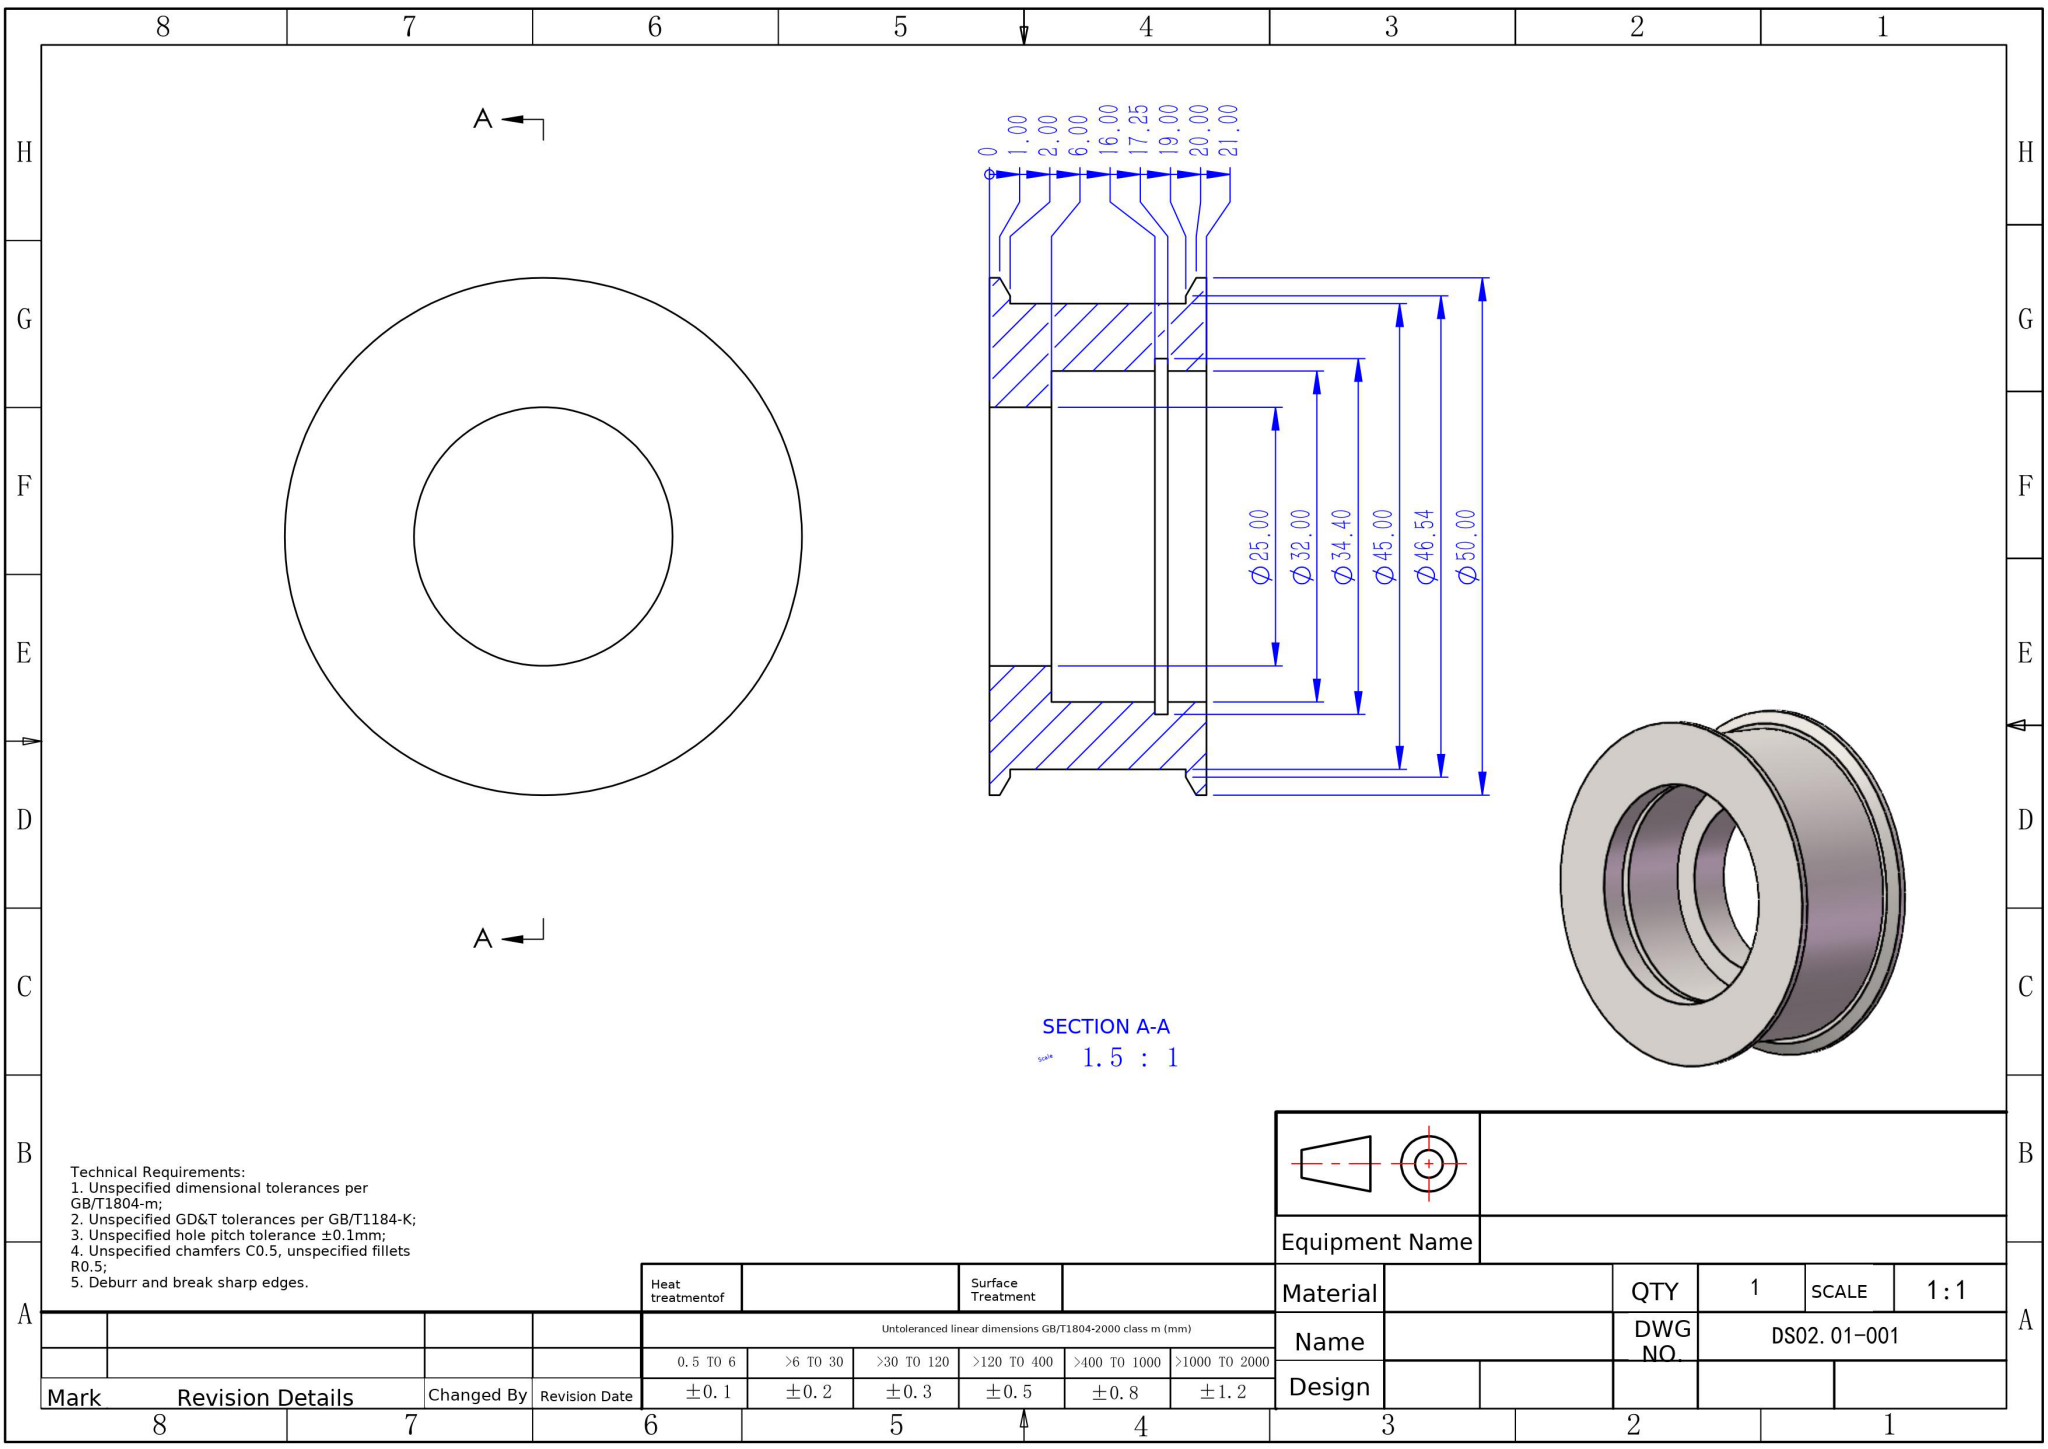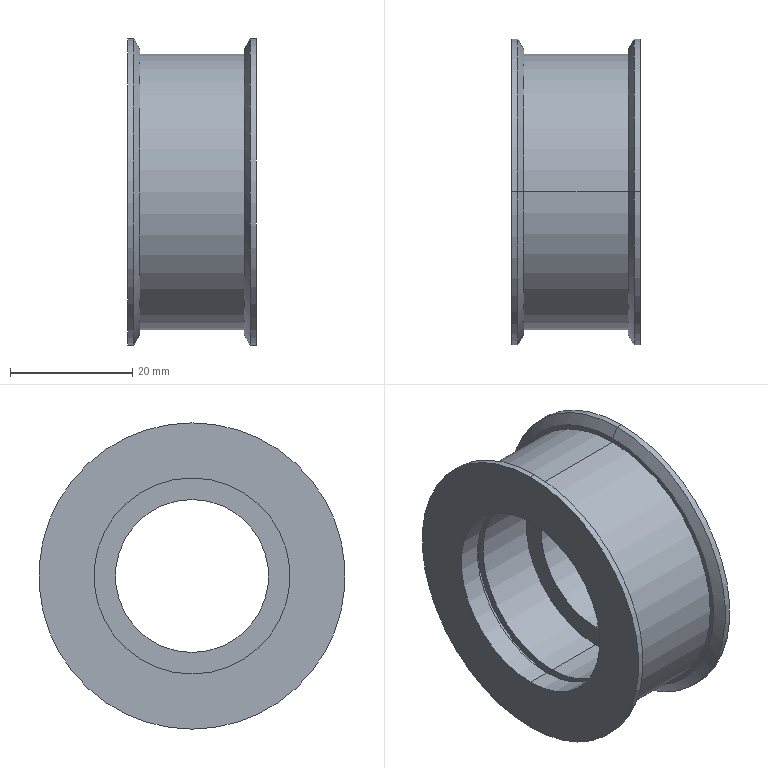Part | NX | mm | 1 solid | 25 faces | box 21 x 50 x 50 mm | volume 19460 mm3 | cylinder 14 | plane 7 | cone 4 | commonest cylinder face diameters 32 x4 50 x4 34.4 x2 45 x2 25 x2
STEP:
#1=CARTESIAN_POINT('',(-17.25,0.,17.2));
#2=VERTEX_POINT('',#1);
#3=CARTESIAN_POINT('',(-17.25,0.,-17.2));
#4=VERTEX_POINT('',#3);
#5=CARTESIAN_POINT('',(-17.25,0.,0.));
#6=DIRECTION('',(1.,0.,0.));
#7=DIRECTION('',(0.,0.,-1.));
#8=AXIS2_PLACEMENT_3D('',#5,#6,#7);
#9=CIRCLE('',#8,17.2);
#10=EDGE_CURVE('',#2,#4,#9,.T.);
#11=ORIENTED_EDGE('',*,*,#10,.F.);
#12=CARTESIAN_POINT('',(-16.,0.,17.2));
#13=VERTEX_POINT('',#12);
#14=CARTESIAN_POINT('',(0.,0.,17.2));
#15=DIRECTION('',(1.,0.,0.));
#16=VECTOR('',#15,1000.);
#17=LINE('',#14,#16);
#18=EDGE_CURVE('',#2,#13,#17,.T.);
#19=ORIENTED_EDGE('',*,*,#18,.T.);
#20=CARTESIAN_POINT('',(-16.,0.,-17.2));
#21=VERTEX_POINT('',#20);
#22=CARTESIAN_POINT('',(-16.,0.,0.));
#23=DIRECTION('',(1.,0.,0.));
#24=DIRECTION('',(0.,0.,-1.));
#25=AXIS2_PLACEMENT_3D('',#22,#23,#24);
#26=CIRCLE('',#25,17.2);
#27=EDGE_CURVE('',#13,#21,#26,.T.);
#28=ORIENTED_EDGE('',*,*,#27,.T.);
#29=CARTESIAN_POINT('',(0.,0.,-17.2));
#30=DIRECTION('',(1.,0.,0.));
#31=VECTOR('',#30,1000.);
#32=LINE('',#29,#31);
#33=EDGE_CURVE('',#4,#21,#32,.T.);
#34=ORIENTED_EDGE('',*,*,#33,.F.);
#35=EDGE_LOOP('',(#11,#19,#28,#34));
#36=FACE_OUTER_BOUND('',#35,.T.);
#37=CARTESIAN_POINT('',(0.,0.,0.));
#38=DIRECTION('',(1.,0.,0.));
#39=DIRECTION('',(0.,0.,-1.));
#40=AXIS2_PLACEMENT_3D('',#37,#38,#39);
#41=CYLINDRICAL_SURFACE('',#40,17.2);
#42=ADVANCED_FACE('',(#36),#41,.F.);
#43=CARTESIAN_POINT('',(-6.,0.,-16.));
#44=VERTEX_POINT('',#43);
#45=CARTESIAN_POINT('',(-6.,0.,16.));
#46=VERTEX_POINT('',#45);
#47=CARTESIAN_POINT('',(-6.,0.,0.));
#48=DIRECTION('',(-1.,0.,0.));
#49=DIRECTION('',(0.,0.,1.));
#50=AXIS2_PLACEMENT_3D('',#47,#48,#49);
#51=CIRCLE('',#50,16.);
#52=EDGE_CURVE('',#44,#46,#51,.T.);
#53=ORIENTED_EDGE('',*,*,#52,.F.);
#54=CARTESIAN_POINT('',(-16.,0.,-16.));
#55=VERTEX_POINT('',#54);
#56=CARTESIAN_POINT('',(-6.,0.,-16.));
#57=DIRECTION('',(-1.,0.,0.));
#58=VECTOR('',#57,1000.);
#59=LINE('',#56,#58);
#60=EDGE_CURVE('',#44,#55,#59,.T.);
#61=ORIENTED_EDGE('',*,*,#60,.T.);
#62=CARTESIAN_POINT('',(-16.,0.,16.));
#63=VERTEX_POINT('',#62);
#64=CARTESIAN_POINT('',(-16.,0.,0.));
#65=DIRECTION('',(1.,0.,0.));
#66=DIRECTION('',(0.,0.,-1.));
#67=AXIS2_PLACEMENT_3D('',#64,#65,#66);
#68=CIRCLE('',#67,16.);
#69=EDGE_CURVE('',#63,#55,#68,.T.);
#70=ORIENTED_EDGE('',*,*,#69,.F.);
#71=CARTESIAN_POINT('',(-6.,0.,16.));
#72=DIRECTION('',(-1.,0.,0.));
#73=VECTOR('',#72,1000.);
#74=LINE('',#71,#73);
#75=EDGE_CURVE('',#46,#63,#74,.T.);
#76=ORIENTED_EDGE('',*,*,#75,.F.);
#77=EDGE_LOOP('',(#53,#61,#70,#76));
#78=FACE_OUTER_BOUND('',#77,.T.);
#79=CARTESIAN_POINT('',(-6.,0.,0.));
#80=DIRECTION('',(-1.,0.,0.));
#81=DIRECTION('',(0.,0.,1.));
#82=AXIS2_PLACEMENT_3D('',#79,#80,#81);
#83=CYLINDRICAL_SURFACE('',#82,16.);
#84=ADVANCED_FACE('',(#78),#83,.F.);
#85=CARTESIAN_POINT('',(-21.,0.,-25.));
#86=VERTEX_POINT('',#85);
#87=CARTESIAN_POINT('',(-21.,0.,25.));
#88=VERTEX_POINT('',#87);
#89=CARTESIAN_POINT('',(-21.,0.,0.));
#90=DIRECTION('',(1.,0.,0.));
#91=DIRECTION('',(0.,0.,-1.));
#92=AXIS2_PLACEMENT_3D('',#89,#90,#91);
#93=CIRCLE('',#92,25.);
#94=EDGE_CURVE('',#86,#88,#93,.T.);
#95=ORIENTED_EDGE('',*,*,#94,.T.);
#96=CARTESIAN_POINT('',(-20.,0.,25.));
#97=VERTEX_POINT('',#96);
#98=CARTESIAN_POINT('',(0.,0.,25.));
#99=DIRECTION('',(1.,0.,0.));
#100=VECTOR('',#99,1000.);
#101=LINE('',#98,#100);
#102=EDGE_CURVE('',#88,#97,#101,.T.);
#103=ORIENTED_EDGE('',*,*,#102,.T.);
#104=CARTESIAN_POINT('',(-20.,0.,-25.));
#105=VERTEX_POINT('',#104);
#106=CARTESIAN_POINT('',(-20.,0.,0.));
#107=DIRECTION('',(1.,0.,0.));
#108=DIRECTION('',(0.,0.,-1.));
#109=AXIS2_PLACEMENT_3D('',#106,#107,#108);
#110=CIRCLE('',#109,25.);
#111=EDGE_CURVE('',#105,#97,#110,.T.);
#112=ORIENTED_EDGE('',*,*,#111,.F.);
#113=CARTESIAN_POINT('',(0.,0.,-25.));
#114=DIRECTION('',(1.,0.,0.));
#115=VECTOR('',#114,1000.);
#116=LINE('',#113,#115);
#117=EDGE_CURVE('',#86,#105,#116,.T.);
#118=ORIENTED_EDGE('',*,*,#117,.F.);
#119=EDGE_LOOP('',(#95,#103,#112,#118));
#120=FACE_OUTER_BOUND('',#119,.T.);
#121=CARTESIAN_POINT('',(0.,0.,0.));
#122=DIRECTION('',(1.,0.,0.));
#123=DIRECTION('',(0.,0.,-1.));
#124=AXIS2_PLACEMENT_3D('',#121,#122,#123);
#125=CYLINDRICAL_SURFACE('',#124,25.);
#126=ADVANCED_FACE('',(#120),#125,.T.);
#127=CARTESIAN_POINT('',(-19.,0.,-23.268));
#128=VERTEX_POINT('',#127);
#129=CARTESIAN_POINT('',(-19.,0.,23.268));
#130=VERTEX_POINT('',#129);
#131=CARTESIAN_POINT('',(-19.,0.,0.));
#132=DIRECTION('',(1.,0.,0.));
#133=DIRECTION('',(0.,0.,-1.));
#134=AXIS2_PLACEMENT_3D('',#131,#132,#133);
#135=CIRCLE('',#134,23.268);
#136=EDGE_CURVE('',#128,#130,#135,.T.);
#137=ORIENTED_EDGE('',*,*,#136,.F.);
#138=CARTESIAN_POINT('',(-19.,0.,-23.268));
#139=DIRECTION('',(-0.5,0.,-0.866));
#140=VECTOR('',#139,1000.);
#141=LINE('',#138,#140);
#142=EDGE_CURVE('',#128,#105,#141,.T.);
#143=ORIENTED_EDGE('',*,*,#142,.T.);
#144=ORIENTED_EDGE('',*,*,#111,.T.);
#145=CARTESIAN_POINT('',(-19.,0.,23.268));
#146=DIRECTION('',(-0.5,0.,0.866));
#147=VECTOR('',#146,1000.);
#148=LINE('',#145,#147);
#149=EDGE_CURVE('',#130,#97,#148,.T.);
#150=ORIENTED_EDGE('',*,*,#149,.F.);
#151=EDGE_LOOP('',(#137,#143,#144,#150));
#152=FACE_OUTER_BOUND('',#151,.T.);
#153=CARTESIAN_POINT('',(-19.,0.,0.));
#154=DIRECTION('',(-1.,0.,0.));
#155=DIRECTION('',(0.,0.,1.));
#156=AXIS2_PLACEMENT_3D('',#153,#154,#155);
#157=CONICAL_SURFACE('',#156,23.268,1.047);
#158=ADVANCED_FACE('',(#152),#157,.T.);
#159=CARTESIAN_POINT('',(-19.,0.,-22.5));
#160=VERTEX_POINT('',#159);
#161=CARTESIAN_POINT('',(-19.,0.,22.5));
#162=VERTEX_POINT('',#161);
#163=CARTESIAN_POINT('',(-19.,0.,0.));
#164=DIRECTION('',(1.,0.,0.));
#165=DIRECTION('',(0.,0.,-1.));
#166=AXIS2_PLACEMENT_3D('',#163,#164,#165);
#167=CIRCLE('',#166,22.5);
#168=EDGE_CURVE('',#160,#162,#167,.T.);
#169=ORIENTED_EDGE('',*,*,#168,.T.);
#170=CARTESIAN_POINT('',(-2.,0.,22.5));
#171=VERTEX_POINT('',#170);
#172=CARTESIAN_POINT('',(0.,0.,22.5));
#173=DIRECTION('',(1.,0.,0.));
#174=VECTOR('',#173,1000.);
#175=LINE('',#172,#174);
#176=EDGE_CURVE('',#162,#171,#175,.T.);
#177=ORIENTED_EDGE('',*,*,#176,.T.);
#178=CARTESIAN_POINT('',(-2.,0.,-22.5));
#179=VERTEX_POINT('',#178);
#180=CARTESIAN_POINT('',(-2.,0.,0.));
#181=DIRECTION('',(1.,0.,0.));
#182=DIRECTION('',(0.,0.,-1.));
#183=AXIS2_PLACEMENT_3D('',#180,#181,#182);
#184=CIRCLE('',#183,22.5);
#185=EDGE_CURVE('',#179,#171,#184,.T.);
#186=ORIENTED_EDGE('',*,*,#185,.F.);
#187=CARTESIAN_POINT('',(0.,0.,-22.5));
#188=DIRECTION('',(1.,0.,0.));
#189=VECTOR('',#188,1000.);
#190=LINE('',#187,#189);
#191=EDGE_CURVE('',#160,#179,#190,.T.);
#192=ORIENTED_EDGE('',*,*,#191,.F.);
#193=EDGE_LOOP('',(#169,#177,#186,#192));
#194=FACE_OUTER_BOUND('',#193,.T.);
#195=CARTESIAN_POINT('',(0.,0.,0.));
#196=DIRECTION('',(1.,0.,0.));
#197=DIRECTION('',(0.,0.,-1.));
#198=AXIS2_PLACEMENT_3D('',#195,#196,#197);
#199=CYLINDRICAL_SURFACE('',#198,22.5);
#200=ADVANCED_FACE('',(#194),#199,.T.);
#201=CARTESIAN_POINT('',(-2.,0.,-23.268));
#202=VERTEX_POINT('',#201);
#203=CARTESIAN_POINT('',(-2.,0.,23.268));
#204=VERTEX_POINT('',#203);
#205=CARTESIAN_POINT('',(-2.,0.,0.));
#206=DIRECTION('',(1.,0.,0.));
#207=DIRECTION('',(0.,0.,-1.));
#208=AXIS2_PLACEMENT_3D('',#205,#206,#207);
#209=CIRCLE('',#208,23.268);
#210=EDGE_CURVE('',#202,#204,#209,.T.);
#211=ORIENTED_EDGE('',*,*,#210,.T.);
#212=CARTESIAN_POINT('',(-1.,0.,25.));
#213=VERTEX_POINT('',#212);
#214=CARTESIAN_POINT('',(-1.,0.,25.));
#215=DIRECTION('',(0.5,0.,0.866));
#216=VECTOR('',#215,1000.);
#217=LINE('',#214,#216);
#218=EDGE_CURVE('',#204,#213,#217,.T.);
#219=ORIENTED_EDGE('',*,*,#218,.T.);
#220=CARTESIAN_POINT('',(-1.,0.,-25.));
#221=VERTEX_POINT('',#220);
#222=CARTESIAN_POINT('',(-1.,0.,0.));
#223=DIRECTION('',(1.,0.,0.));
#224=DIRECTION('',(0.,0.,-1.));
#225=AXIS2_PLACEMENT_3D('',#222,#223,#224);
#226=CIRCLE('',#225,25.);
#227=EDGE_CURVE('',#221,#213,#226,.T.);
#228=ORIENTED_EDGE('',*,*,#227,.F.);
#229=CARTESIAN_POINT('',(-1.,0.,-25.));
#230=DIRECTION('',(0.5,0.,-0.866));
#231=VECTOR('',#230,1000.);
#232=LINE('',#229,#231);
#233=EDGE_CURVE('',#202,#221,#232,.T.);
#234=ORIENTED_EDGE('',*,*,#233,.F.);
#235=EDGE_LOOP('',(#211,#219,#228,#234));
#236=FACE_OUTER_BOUND('',#235,.T.);
#237=CARTESIAN_POINT('',(-1.,0.,0.));
#238=DIRECTION('',(1.,0.,0.));
#239=DIRECTION('',(0.,0.,-1.));
#240=AXIS2_PLACEMENT_3D('',#237,#238,#239);
#241=CONICAL_SURFACE('',#240,25.,1.047);
#242=ADVANCED_FACE('',(#236),#241,.T.);
#243=ORIENTED_EDGE('',*,*,#227,.T.);
#244=CARTESIAN_POINT('',(-0.,0.,25.));
#245=VERTEX_POINT('',#244);
#246=CARTESIAN_POINT('',(0.,0.,25.));
#247=DIRECTION('',(1.,0.,0.));
#248=VECTOR('',#247,1000.);
#249=LINE('',#246,#248);
#250=EDGE_CURVE('',#213,#245,#249,.T.);
#251=ORIENTED_EDGE('',*,*,#250,.T.);
#252=CARTESIAN_POINT('',(-0.,0.,-25.));
#253=VERTEX_POINT('',#252);
#254=CARTESIAN_POINT('',(-0.,0.,0.));
#255=DIRECTION('',(1.,0.,0.));
#256=DIRECTION('',(0.,0.,-1.));
#257=AXIS2_PLACEMENT_3D('',#254,#255,#256);
#258=CIRCLE('',#257,25.);
#259=EDGE_CURVE('',#253,#245,#258,.T.);
#260=ORIENTED_EDGE('',*,*,#259,.F.);
#261=CARTESIAN_POINT('',(0.,0.,-25.));
#262=DIRECTION('',(1.,0.,0.));
#263=VECTOR('',#262,1000.);
#264=LINE('',#261,#263);
#265=EDGE_CURVE('',#221,#253,#264,.T.);
#266=ORIENTED_EDGE('',*,*,#265,.F.);
#267=EDGE_LOOP('',(#243,#251,#260,#266));
#268=FACE_OUTER_BOUND('',#267,.T.);
#269=CARTESIAN_POINT('',(0.,0.,0.));
#270=DIRECTION('',(1.,0.,0.));
#271=DIRECTION('',(0.,0.,-1.));
#272=AXIS2_PLACEMENT_3D('',#269,#270,#271);
#273=CYLINDRICAL_SURFACE('',#272,25.);
#274=ADVANCED_FACE('',(#268),#273,.T.);
#275=CARTESIAN_POINT('',(-6.,0.,-12.5));
#276=VERTEX_POINT('',#275);
#277=CARTESIAN_POINT('',(-6.,0.,12.5));
#278=VERTEX_POINT('',#277);
#279=CARTESIAN_POINT('',(-6.,0.,0.));
#280=DIRECTION('',(-1.,0.,0.));
#281=DIRECTION('',(0.,0.,1.));
#282=AXIS2_PLACEMENT_3D('',#279,#280,#281);
#283=CIRCLE('',#282,12.5);
#284=EDGE_CURVE('',#276,#278,#283,.T.);
#285=ORIENTED_EDGE('',*,*,#284,.T.);
#286=CARTESIAN_POINT('',(0.,0.,12.5));
#287=VERTEX_POINT('',#286);
#288=CARTESIAN_POINT('',(0.,0.,12.5));
#289=DIRECTION('',(1.,0.,0.));
#290=VECTOR('',#289,1000.);
#291=LINE('',#288,#290);
#292=EDGE_CURVE('',#278,#287,#291,.T.);
#293=ORIENTED_EDGE('',*,*,#292,.T.);
#294=CARTESIAN_POINT('',(0.,0.,-12.5));
#295=VERTEX_POINT('',#294);
#296=CARTESIAN_POINT('',(0.,0.,0.));
#297=DIRECTION('',(1.,0.,0.));
#298=DIRECTION('',(0.,0.,-1.));
#299=AXIS2_PLACEMENT_3D('',#296,#297,#298);
#300=CIRCLE('',#299,12.5);
#301=EDGE_CURVE('',#287,#295,#300,.T.);
#302=ORIENTED_EDGE('',*,*,#301,.T.);
#303=CARTESIAN_POINT('',(0.,0.,-12.5));
#304=DIRECTION('',(1.,0.,0.));
#305=VECTOR('',#304,1000.);
#306=LINE('',#303,#305);
#307=EDGE_CURVE('',#276,#295,#306,.T.);
#308=ORIENTED_EDGE('',*,*,#307,.F.);
#309=EDGE_LOOP('',(#285,#293,#302,#308));
#310=FACE_OUTER_BOUND('',#309,.T.);
#311=CARTESIAN_POINT('',(0.,0.,0.));
#312=DIRECTION('',(1.,0.,0.));
#313=DIRECTION('',(0.,0.,-1.));
#314=AXIS2_PLACEMENT_3D('',#311,#312,#313);
#315=CYLINDRICAL_SURFACE('',#314,12.5);
#316=ADVANCED_FACE('',(#310),#315,.F.);
#317=CARTESIAN_POINT('',(-17.25,0.,16.));
#318=VERTEX_POINT('',#317);
#319=CARTESIAN_POINT('',(-17.25,0.,-16.));
#320=VERTEX_POINT('',#319);
#321=CARTESIAN_POINT('',(-17.25,0.,0.));
#322=DIRECTION('',(1.,0.,0.));
#323=DIRECTION('',(0.,0.,-1.));
#324=AXIS2_PLACEMENT_3D('',#321,#322,#323);
#325=CIRCLE('',#324,16.);
#326=EDGE_CURVE('',#318,#320,#325,.T.);
#327=ORIENTED_EDGE('',*,*,#326,.T.);
#328=CARTESIAN_POINT('',(-21.,0.,-16.));
#329=VERTEX_POINT('',#328);
#330=CARTESIAN_POINT('',(-6.,0.,-16.));
#331=DIRECTION('',(-1.,0.,0.));
#332=VECTOR('',#331,1000.);
#333=LINE('',#330,#332);
#334=EDGE_CURVE('',#320,#329,#333,.T.);
#335=ORIENTED_EDGE('',*,*,#334,.T.);
#336=CARTESIAN_POINT('',(-21.,0.,16.));
#337=VERTEX_POINT('',#336);
#338=CARTESIAN_POINT('',(-21.,0.,0.));
#339=DIRECTION('',(-1.,0.,0.));
#340=DIRECTION('',(0.,0.,1.));
#341=AXIS2_PLACEMENT_3D('',#338,#339,#340);
#342=CIRCLE('',#341,16.);
#343=EDGE_CURVE('',#329,#337,#342,.T.);
#344=ORIENTED_EDGE('',*,*,#343,.T.);
#345=CARTESIAN_POINT('',(-6.,0.,16.));
#346=DIRECTION('',(-1.,0.,0.));
#347=VECTOR('',#346,1000.);
#348=LINE('',#345,#347);
#349=EDGE_CURVE('',#318,#337,#348,.T.);
#350=ORIENTED_EDGE('',*,*,#349,.F.);
#351=EDGE_LOOP('',(#327,#335,#344,#350));
#352=FACE_OUTER_BOUND('',#351,.T.);
#353=CARTESIAN_POINT('',(-6.,0.,0.));
#354=DIRECTION('',(-1.,0.,0.));
#355=DIRECTION('',(0.,0.,1.));
#356=AXIS2_PLACEMENT_3D('',#353,#354,#355);
#357=CYLINDRICAL_SURFACE('',#356,16.);
#358=ADVANCED_FACE('',(#352),#357,.F.);
#359=ORIENTED_EDGE('',*,*,#334,.F.);
#360=CARTESIAN_POINT('',(-17.25,0.,0.));
#361=DIRECTION('',(1.,0.,0.));
#362=DIRECTION('',(0.,0.,-1.));
#363=AXIS2_PLACEMENT_3D('',#360,#361,#362);
#364=CIRCLE('',#363,16.);
#365=EDGE_CURVE('',#320,#318,#364,.T.);
#366=ORIENTED_EDGE('',*,*,#365,.T.);
#367=ORIENTED_EDGE('',*,*,#349,.T.);
#368=CARTESIAN_POINT('',(-21.,0.,0.));
#369=DIRECTION('',(-1.,0.,0.));
#370=DIRECTION('',(0.,0.,1.));
#371=AXIS2_PLACEMENT_3D('',#368,#369,#370);
#372=CIRCLE('',#371,16.);
#373=EDGE_CURVE('',#337,#329,#372,.T.);
#374=ORIENTED_EDGE('',*,*,#373,.T.);
#375=EDGE_LOOP('',(#359,#366,#367,#374));
#376=FACE_OUTER_BOUND('',#375,.T.);
#377=CARTESIAN_POINT('',(-6.,0.,0.));
#378=DIRECTION('',(-1.,0.,0.));
#379=DIRECTION('',(0.,0.,1.));
#380=AXIS2_PLACEMENT_3D('',#377,#378,#379);
#381=CYLINDRICAL_SURFACE('',#380,16.);
#382=ADVANCED_FACE('',(#376),#381,.F.);
#383=ORIENTED_EDGE('',*,*,#292,.F.);
#384=CARTESIAN_POINT('',(-6.,0.,0.));
#385=DIRECTION('',(-1.,0.,0.));
#386=DIRECTION('',(0.,0.,1.));
#387=AXIS2_PLACEMENT_3D('',#384,#385,#386);
#388=CIRCLE('',#387,12.5);
#389=EDGE_CURVE('',#278,#276,#388,.T.);
#390=ORIENTED_EDGE('',*,*,#389,.T.);
#391=ORIENTED_EDGE('',*,*,#307,.T.);
#392=CARTESIAN_POINT('',(0.,0.,0.));
#393=DIRECTION('',(1.,0.,0.));
#394=DIRECTION('',(0.,0.,-1.));
#395=AXIS2_PLACEMENT_3D('',#392,#393,#394);
#396=CIRCLE('',#395,12.5);
#397=EDGE_CURVE('',#295,#287,#396,.T.);
#398=ORIENTED_EDGE('',*,*,#397,.T.);
#399=EDGE_LOOP('',(#383,#390,#391,#398));
#400=FACE_OUTER_BOUND('',#399,.T.);
#401=CARTESIAN_POINT('',(0.,0.,0.));
#402=DIRECTION('',(1.,0.,0.));
#403=DIRECTION('',(0.,0.,-1.));
#404=AXIS2_PLACEMENT_3D('',#401,#402,#403);
#405=CYLINDRICAL_SURFACE('',#404,12.5);
#406=ADVANCED_FACE('',(#400),#405,.F.);
#407=ORIENTED_EDGE('',*,*,#259,.T.);
#408=CARTESIAN_POINT('',(-0.,0.,0.));
#409=DIRECTION('',(1.,0.,0.));
#410=DIRECTION('',(0.,0.,-1.));
#411=AXIS2_PLACEMENT_3D('',#408,#409,#410);
#412=CIRCLE('',#411,25.);
#413=EDGE_CURVE('',#245,#253,#412,.T.);
#414=ORIENTED_EDGE('',*,*,#413,.T.);
#415=EDGE_LOOP('',(#407,#414));
#416=FACE_OUTER_BOUND('',#415,.T.);
#417=ORIENTED_EDGE('',*,*,#397,.F.);
#418=ORIENTED_EDGE('',*,*,#301,.F.);
#419=EDGE_LOOP('',(#417,#418));
#420=FACE_BOUND('',#419,.T.);
#421=CARTESIAN_POINT('',(-0.,12.5,0.));
#422=DIRECTION('',(1.,0.,0.));
#423=DIRECTION('',(0.,0.,-1.));
#424=AXIS2_PLACEMENT_3D('',#421,#422,#423);
#425=PLANE('',#424);
#426=ADVANCED_FACE('',(#416,#420),#425,.T.);
#427=ORIENTED_EDGE('',*,*,#250,.F.);
#428=CARTESIAN_POINT('',(-1.,0.,0.));
#429=DIRECTION('',(1.,0.,0.));
#430=DIRECTION('',(0.,0.,-1.));
#431=AXIS2_PLACEMENT_3D('',#428,#429,#430);
#432=CIRCLE('',#431,25.);
#433=EDGE_CURVE('',#213,#221,#432,.T.);
#434=ORIENTED_EDGE('',*,*,#433,.T.);
#435=ORIENTED_EDGE('',*,*,#265,.T.);
#436=ORIENTED_EDGE('',*,*,#413,.F.);
#437=EDGE_LOOP('',(#427,#434,#435,#436));
#438=FACE_OUTER_BOUND('',#437,.T.);
#439=CARTESIAN_POINT('',(0.,0.,0.));
#440=DIRECTION('',(1.,0.,0.));
#441=DIRECTION('',(0.,0.,-1.));
#442=AXIS2_PLACEMENT_3D('',#439,#440,#441);
#443=CYLINDRICAL_SURFACE('',#442,25.);
#444=ADVANCED_FACE('',(#438),#443,.T.);
#445=ORIENTED_EDGE('',*,*,#218,.F.);
#446=CARTESIAN_POINT('',(-2.,0.,0.));
#447=DIRECTION('',(1.,0.,0.));
#448=DIRECTION('',(0.,0.,-1.));
#449=AXIS2_PLACEMENT_3D('',#446,#447,#448);
#450=CIRCLE('',#449,23.268);
#451=EDGE_CURVE('',#204,#202,#450,.T.);
#452=ORIENTED_EDGE('',*,*,#451,.T.);
#453=ORIENTED_EDGE('',*,*,#233,.T.);
#454=ORIENTED_EDGE('',*,*,#433,.F.);
#455=EDGE_LOOP('',(#445,#452,#453,#454));
#456=FACE_OUTER_BOUND('',#455,.T.);
#457=CARTESIAN_POINT('',(-1.,0.,0.));
#458=DIRECTION('',(1.,0.,0.));
#459=DIRECTION('',(0.,0.,-1.));
#460=AXIS2_PLACEMENT_3D('',#457,#458,#459);
#461=CONICAL_SURFACE('',#460,25.,1.047);
#462=ADVANCED_FACE('',(#456),#461,.T.);
#463=ORIENTED_EDGE('',*,*,#185,.T.);
#464=CARTESIAN_POINT('',(-2.,0.,0.));
#465=DIRECTION('',(1.,0.,0.));
#466=DIRECTION('',(0.,0.,-1.));
#467=AXIS2_PLACEMENT_3D('',#464,#465,#466);
#468=CIRCLE('',#467,22.5);
#469=EDGE_CURVE('',#171,#179,#468,.T.);
#470=ORIENTED_EDGE('',*,*,#469,.T.);
#471=EDGE_LOOP('',(#463,#470));
#472=FACE_BOUND('',#471,.T.);
#473=ORIENTED_EDGE('',*,*,#210,.F.);
#474=ORIENTED_EDGE('',*,*,#451,.F.);
#475=EDGE_LOOP('',(#473,#474));
#476=FACE_OUTER_BOUND('',#475,.T.);
#477=CARTESIAN_POINT('',(-2.,23.268,0.));
#478=DIRECTION('',(-1.,0.,0.));
#479=DIRECTION('',(0.,0.,1.));
#480=AXIS2_PLACEMENT_3D('',#477,#478,#479);
#481=PLANE('',#480);
#482=ADVANCED_FACE('',(#472,#476),#481,.T.);
#483=ORIENTED_EDGE('',*,*,#176,.F.);
#484=CARTESIAN_POINT('',(-19.,0.,0.));
#485=DIRECTION('',(1.,0.,0.));
#486=DIRECTION('',(0.,0.,-1.));
#487=AXIS2_PLACEMENT_3D('',#484,#485,#486);
#488=CIRCLE('',#487,22.5);
#489=EDGE_CURVE('',#162,#160,#488,.T.);
#490=ORIENTED_EDGE('',*,*,#489,.T.);
#491=ORIENTED_EDGE('',*,*,#191,.T.);
#492=ORIENTED_EDGE('',*,*,#469,.F.);
#493=EDGE_LOOP('',(#483,#490,#491,#492));
#494=FACE_OUTER_BOUND('',#493,.T.);
#495=CARTESIAN_POINT('',(0.,0.,0.));
#496=DIRECTION('',(1.,0.,0.));
#497=DIRECTION('',(0.,0.,-1.));
#498=AXIS2_PLACEMENT_3D('',#495,#496,#497);
#499=CYLINDRICAL_SURFACE('',#498,22.5);
#500=ADVANCED_FACE('',(#494),#499,.T.);
#501=CARTESIAN_POINT('',(-19.,0.,0.));
#502=DIRECTION('',(1.,0.,0.));
#503=DIRECTION('',(0.,0.,-1.));
#504=AXIS2_PLACEMENT_3D('',#501,#502,#503);
#505=CIRCLE('',#504,23.268);
#506=EDGE_CURVE('',#130,#128,#505,.T.);
#507=ORIENTED_EDGE('',*,*,#506,.T.);
#508=ORIENTED_EDGE('',*,*,#136,.T.);
#509=EDGE_LOOP('',(#507,#508));
#510=FACE_OUTER_BOUND('',#509,.T.);
#511=ORIENTED_EDGE('',*,*,#168,.F.);
#512=ORIENTED_EDGE('',*,*,#489,.F.);
#513=EDGE_LOOP('',(#511,#512));
#514=FACE_BOUND('',#513,.T.);
#515=CARTESIAN_POINT('',(-19.,23.268,0.));
#516=DIRECTION('',(1.,0.,0.));
#517=DIRECTION('',(0.,0.,-1.));
#518=AXIS2_PLACEMENT_3D('',#515,#516,#517);
#519=PLANE('',#518);
#520=ADVANCED_FACE('',(#510,#514),#519,.T.);
#521=ORIENTED_EDGE('',*,*,#142,.F.);
#522=ORIENTED_EDGE('',*,*,#506,.F.);
#523=ORIENTED_EDGE('',*,*,#149,.T.);
#524=CARTESIAN_POINT('',(-20.,0.,0.));
#525=DIRECTION('',(1.,0.,0.));
#526=DIRECTION('',(0.,0.,-1.));
#527=AXIS2_PLACEMENT_3D('',#524,#525,#526);
#528=CIRCLE('',#527,25.);
#529=EDGE_CURVE('',#97,#105,#528,.T.);
#530=ORIENTED_EDGE('',*,*,#529,.T.);
#531=EDGE_LOOP('',(#521,#522,#523,#530));
#532=FACE_OUTER_BOUND('',#531,.T.);
#533=CARTESIAN_POINT('',(-19.,0.,0.));
#534=DIRECTION('',(-1.,0.,0.));
#535=DIRECTION('',(0.,0.,1.));
#536=AXIS2_PLACEMENT_3D('',#533,#534,#535);
#537=CONICAL_SURFACE('',#536,23.268,1.047);
#538=ADVANCED_FACE('',(#532),#537,.T.);
#539=ORIENTED_EDGE('',*,*,#102,.F.);
#540=CARTESIAN_POINT('',(-21.,0.,0.));
#541=DIRECTION('',(1.,0.,0.));
#542=DIRECTION('',(0.,0.,-1.));
#543=AXIS2_PLACEMENT_3D('',#540,#541,#542);
#544=CIRCLE('',#543,25.);
#545=EDGE_CURVE('',#88,#86,#544,.T.);
#546=ORIENTED_EDGE('',*,*,#545,.T.);
#547=ORIENTED_EDGE('',*,*,#117,.T.);
#548=ORIENTED_EDGE('',*,*,#529,.F.);
#549=EDGE_LOOP('',(#539,#546,#547,#548));
#550=FACE_OUTER_BOUND('',#549,.T.);
#551=CARTESIAN_POINT('',(0.,0.,0.));
#552=DIRECTION('',(1.,0.,0.));
#553=DIRECTION('',(0.,0.,-1.));
#554=AXIS2_PLACEMENT_3D('',#551,#552,#553);
#555=CYLINDRICAL_SURFACE('',#554,25.);
#556=ADVANCED_FACE('',(#550),#555,.T.);
#557=ORIENTED_EDGE('',*,*,#373,.F.);
#558=ORIENTED_EDGE('',*,*,#343,.F.);
#559=EDGE_LOOP('',(#557,#558));
#560=FACE_BOUND('',#559,.T.);
#561=ORIENTED_EDGE('',*,*,#94,.F.);
#562=ORIENTED_EDGE('',*,*,#545,.F.);
#563=EDGE_LOOP('',(#561,#562));
#564=FACE_OUTER_BOUND('',#563,.T.);
#565=CARTESIAN_POINT('',(-21.,12.5,0.));
#566=DIRECTION('',(-1.,0.,0.));
#567=DIRECTION('',(0.,0.,1.));
#568=AXIS2_PLACEMENT_3D('',#565,#566,#567);
#569=PLANE('',#568);
#570=ADVANCED_FACE('',(#560,#564),#569,.T.);
#571=ORIENTED_EDGE('',*,*,#60,.F.);
#572=CARTESIAN_POINT('',(-6.,0.,0.));
#573=DIRECTION('',(-1.,0.,0.));
#574=DIRECTION('',(0.,0.,1.));
#575=AXIS2_PLACEMENT_3D('',#572,#573,#574);
#576=CIRCLE('',#575,16.);
#577=EDGE_CURVE('',#46,#44,#576,.T.);
#578=ORIENTED_EDGE('',*,*,#577,.F.);
#579=ORIENTED_EDGE('',*,*,#75,.T.);
#580=CARTESIAN_POINT('',(-16.,0.,0.));
#581=DIRECTION('',(1.,0.,0.));
#582=DIRECTION('',(0.,0.,-1.));
#583=AXIS2_PLACEMENT_3D('',#580,#581,#582);
#584=CIRCLE('',#583,16.);
#585=EDGE_CURVE('',#55,#63,#584,.T.);
#586=ORIENTED_EDGE('',*,*,#585,.F.);
#587=EDGE_LOOP('',(#571,#578,#579,#586));
#588=FACE_OUTER_BOUND('',#587,.T.);
#589=CARTESIAN_POINT('',(-6.,0.,0.));
#590=DIRECTION('',(-1.,0.,0.));
#591=DIRECTION('',(0.,0.,1.));
#592=AXIS2_PLACEMENT_3D('',#589,#590,#591);
#593=CYLINDRICAL_SURFACE('',#592,16.);
#594=ADVANCED_FACE('',(#588),#593,.F.);
#595=ORIENTED_EDGE('',*,*,#284,.F.);
#596=ORIENTED_EDGE('',*,*,#389,.F.);
#597=EDGE_LOOP('',(#595,#596));
#598=FACE_BOUND('',#597,.T.);
#599=ORIENTED_EDGE('',*,*,#577,.T.);
#600=ORIENTED_EDGE('',*,*,#52,.T.);
#601=EDGE_LOOP('',(#599,#600));
#602=FACE_OUTER_BOUND('',#601,.T.);
#603=CARTESIAN_POINT('',(-6.,0.,0.));
#604=DIRECTION('',(-1.,0.,0.));
#605=DIRECTION('',(0.,0.,1.));
#606=AXIS2_PLACEMENT_3D('',#603,#604,#605);
#607=PLANE('',#606);
#608=ADVANCED_FACE('',(#598,#602),#607,.T.);
#609=ORIENTED_EDGE('',*,*,#326,.F.);
#610=ORIENTED_EDGE('',*,*,#365,.F.);
#611=EDGE_LOOP('',(#609,#610));
#612=FACE_BOUND('',#611,.T.);
#613=CARTESIAN_POINT('',(-17.25,0.,0.));
#614=DIRECTION('',(1.,0.,0.));
#615=DIRECTION('',(0.,0.,-1.));
#616=AXIS2_PLACEMENT_3D('',#613,#614,#615);
#617=CIRCLE('',#616,17.2);
#618=EDGE_CURVE('',#4,#2,#617,.T.);
#619=ORIENTED_EDGE('',*,*,#618,.T.);
#620=ORIENTED_EDGE('',*,*,#10,.T.);
#621=EDGE_LOOP('',(#619,#620));
#622=FACE_OUTER_BOUND('',#621,.T.);
#623=CARTESIAN_POINT('',(-17.25,17.2,0.));
#624=DIRECTION('',(-1.,0.,0.));
#625=DIRECTION('',(0.,0.,1.));
#626=AXIS2_PLACEMENT_3D('',#623,#624,#625);
#627=PLANE('',#626);
#628=ADVANCED_FACE('',(#612,#622),#627,.F.);
#629=CARTESIAN_POINT('',(-16.,0.,0.));
#630=DIRECTION('',(1.,0.,0.));
#631=DIRECTION('',(0.,0.,-1.));
#632=AXIS2_PLACEMENT_3D('',#629,#630,#631);
#633=CIRCLE('',#632,17.2);
#634=EDGE_CURVE('',#21,#13,#633,.T.);
#635=ORIENTED_EDGE('',*,*,#634,.F.);
#636=ORIENTED_EDGE('',*,*,#27,.F.);
#637=EDGE_LOOP('',(#635,#636));
#638=FACE_OUTER_BOUND('',#637,.T.);
#639=ORIENTED_EDGE('',*,*,#69,.T.);
#640=ORIENTED_EDGE('',*,*,#585,.T.);
#641=EDGE_LOOP('',(#639,#640));
#642=FACE_BOUND('',#641,.T.);
#643=CARTESIAN_POINT('',(-16.,17.2,0.));
#644=DIRECTION('',(1.,0.,0.));
#645=DIRECTION('',(0.,0.,-1.));
#646=AXIS2_PLACEMENT_3D('',#643,#644,#645);
#647=PLANE('',#646);
#648=ADVANCED_FACE('',(#638,#642),#647,.F.);
#649=ORIENTED_EDGE('',*,*,#18,.F.);
#650=ORIENTED_EDGE('',*,*,#618,.F.);
#651=ORIENTED_EDGE('',*,*,#33,.T.);
#652=ORIENTED_EDGE('',*,*,#634,.T.);
#653=EDGE_LOOP('',(#649,#650,#651,#652));
#654=FACE_OUTER_BOUND('',#653,.T.);
#655=CARTESIAN_POINT('',(0.,0.,0.));
#656=DIRECTION('',(1.,0.,0.));
#657=DIRECTION('',(0.,0.,-1.));
#658=AXIS2_PLACEMENT_3D('',#655,#656,#657);
#659=CYLINDRICAL_SURFACE('',#658,17.2);
#660=ADVANCED_FACE('',(#654),#659,.F.);
#661=CLOSED_SHELL('',(#42,#84,#126,#158,#200,#242,#274,#316,#358,#382,#406,#426,#444,#462,#482,#500,#520,#538,#556,#570,#594,#608,#628,#648,#660));
#662=MANIFOLD_SOLID_BREP('',#661);
#663=CARTESIAN_POINT('',(0.,0.,0.));
#664=DIRECTION('',(0.,0.,1.));
#665=DIRECTION('',(1.,0.,0.));
#666=AXIS2_PLACEMENT_3D('',#663,#664,#665);
#667=(LENGTH_UNIT()NAMED_UNIT(*)SI_UNIT(.MILLI.,.METRE.));
#668=UNCERTAINTY_MEASURE_WITH_UNIT(LENGTH_MEASURE(0.00001),#667,'','');
#669=(NAMED_UNIT(*)PLANE_ANGLE_UNIT()SI_UNIT($,.RADIAN.));
#670=(NAMED_UNIT(*)SI_UNIT($,.STERADIAN.)SOLID_ANGLE_UNIT());
#671=(GEOMETRIC_REPRESENTATION_CONTEXT(3)GLOBAL_UNCERTAINTY_ASSIGNED_CONTEXT((#668))GLOBAL_UNIT_ASSIGNED_CONTEXT((#667,#669,#670))REPRESENTATION_CONTEXT('',''));
#672=ADVANCED_BREP_SHAPE_REPRESENTATION('',(#662,#666),#671);
#673=COLOUR_RGB('',0.7922,0.8196,0.9333);
#674=FILL_AREA_STYLE_COLOUR('',#673);
#675=FILL_AREA_STYLE('',(#674));
#676=SURFACE_STYLE_FILL_AREA(#675);
#677=SURFACE_SIDE_STYLE('',(#676));
#678=SURFACE_STYLE_USAGE(.BOTH.,#677);
#679=PRESENTATION_STYLE_ASSIGNMENT((#678));
#680=STYLED_ITEM('',(#679),#662);
#681=(LENGTH_UNIT()NAMED_UNIT(*)SI_UNIT(.MILLI.,.METRE.));
#682=UNCERTAINTY_MEASURE_WITH_UNIT(LENGTH_MEASURE(0.00001),#681,'','');
#683=(NAMED_UNIT(*)PLANE_ANGLE_UNIT()SI_UNIT($,.RADIAN.));
#684=(NAMED_UNIT(*)SI_UNIT($,.STERADIAN.)SOLID_ANGLE_UNIT());
#685=(GEOMETRIC_REPRESENTATION_CONTEXT(3)GLOBAL_UNCERTAINTY_ASSIGNED_CONTEXT((#682))GLOBAL_UNIT_ASSIGNED_CONTEXT((#681,#683,#684))REPRESENTATION_CONTEXT('',''));
#686=MECHANICAL_DESIGN_GEOMETRIC_PRESENTATION_REPRESENTATION('',(#680),#685);
#687=PRESENTATION_LAYER_ASSIGNMENT('','',(#680));